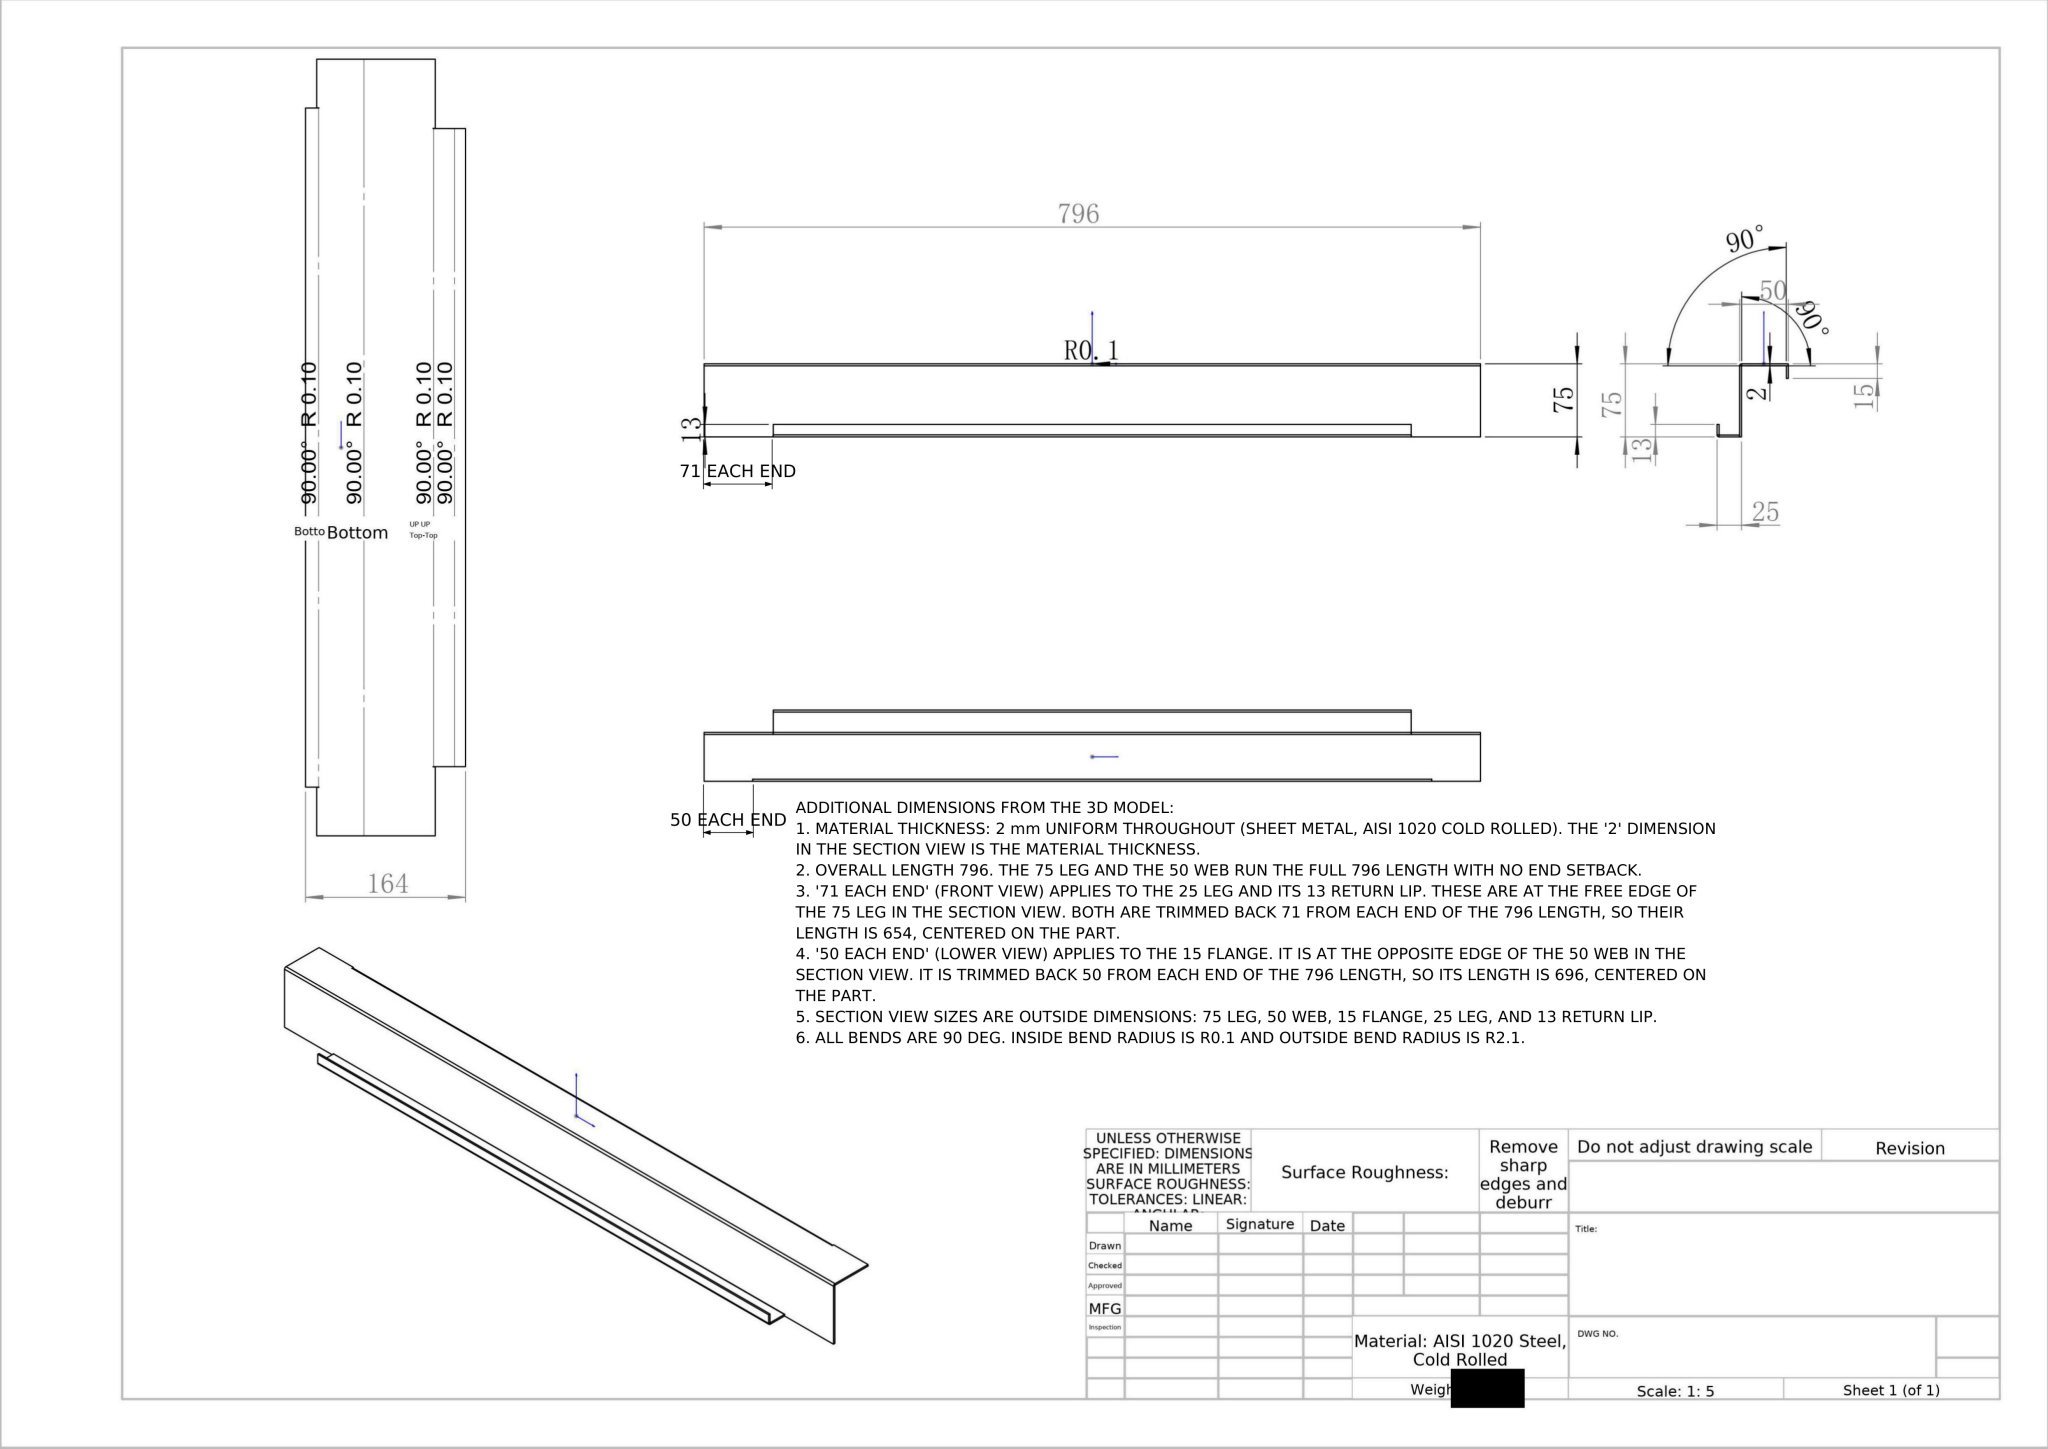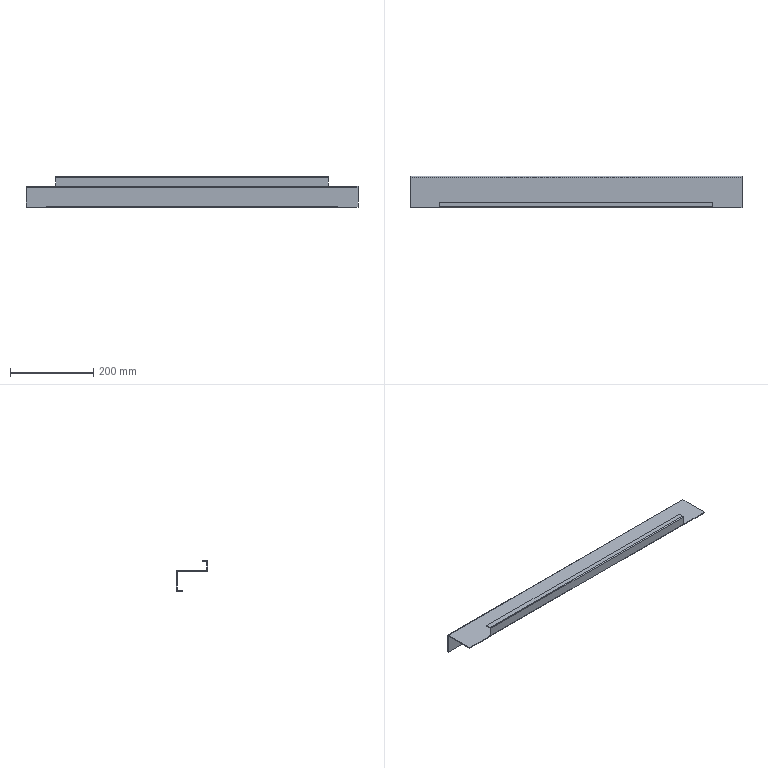Part | NX | mm | Extruded Rectangular Hat Section | 1 solid | 54 faces | box 796 x 75 x 73 mm | volume 255736 mm3 | plane 46 | cylinder 8 | commonest cylinder face diameters 4.2 x4 0.2 x4